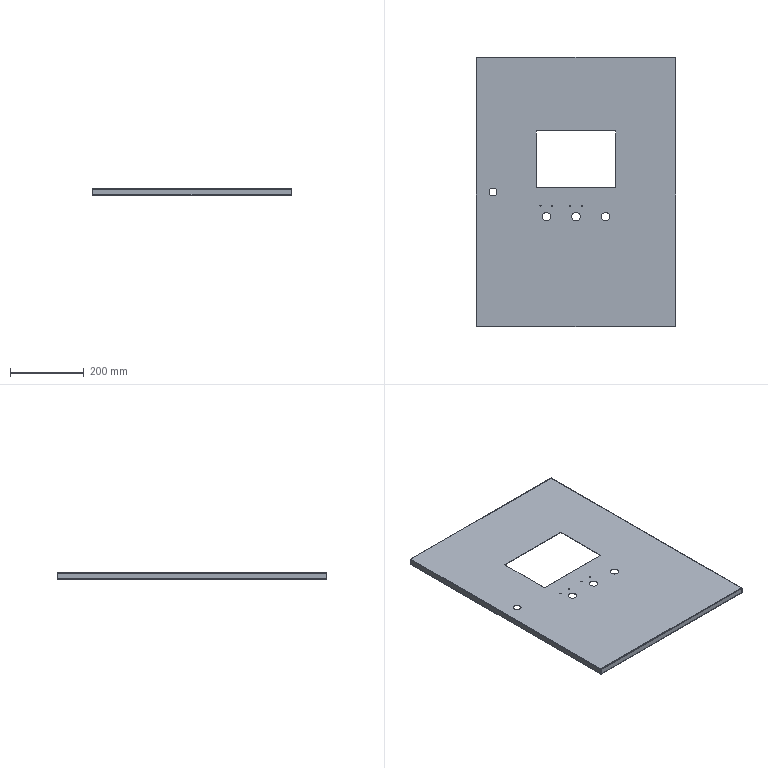Component | SolidWorks | InnerDoor-1 | 1 solid | 104 faces | volume 627735 mm3 | plane 58 | cylinder 34 | spline 12 | commonest cylinder face diameters 3.2 x16 0.2 x8 23 x6 22 x4